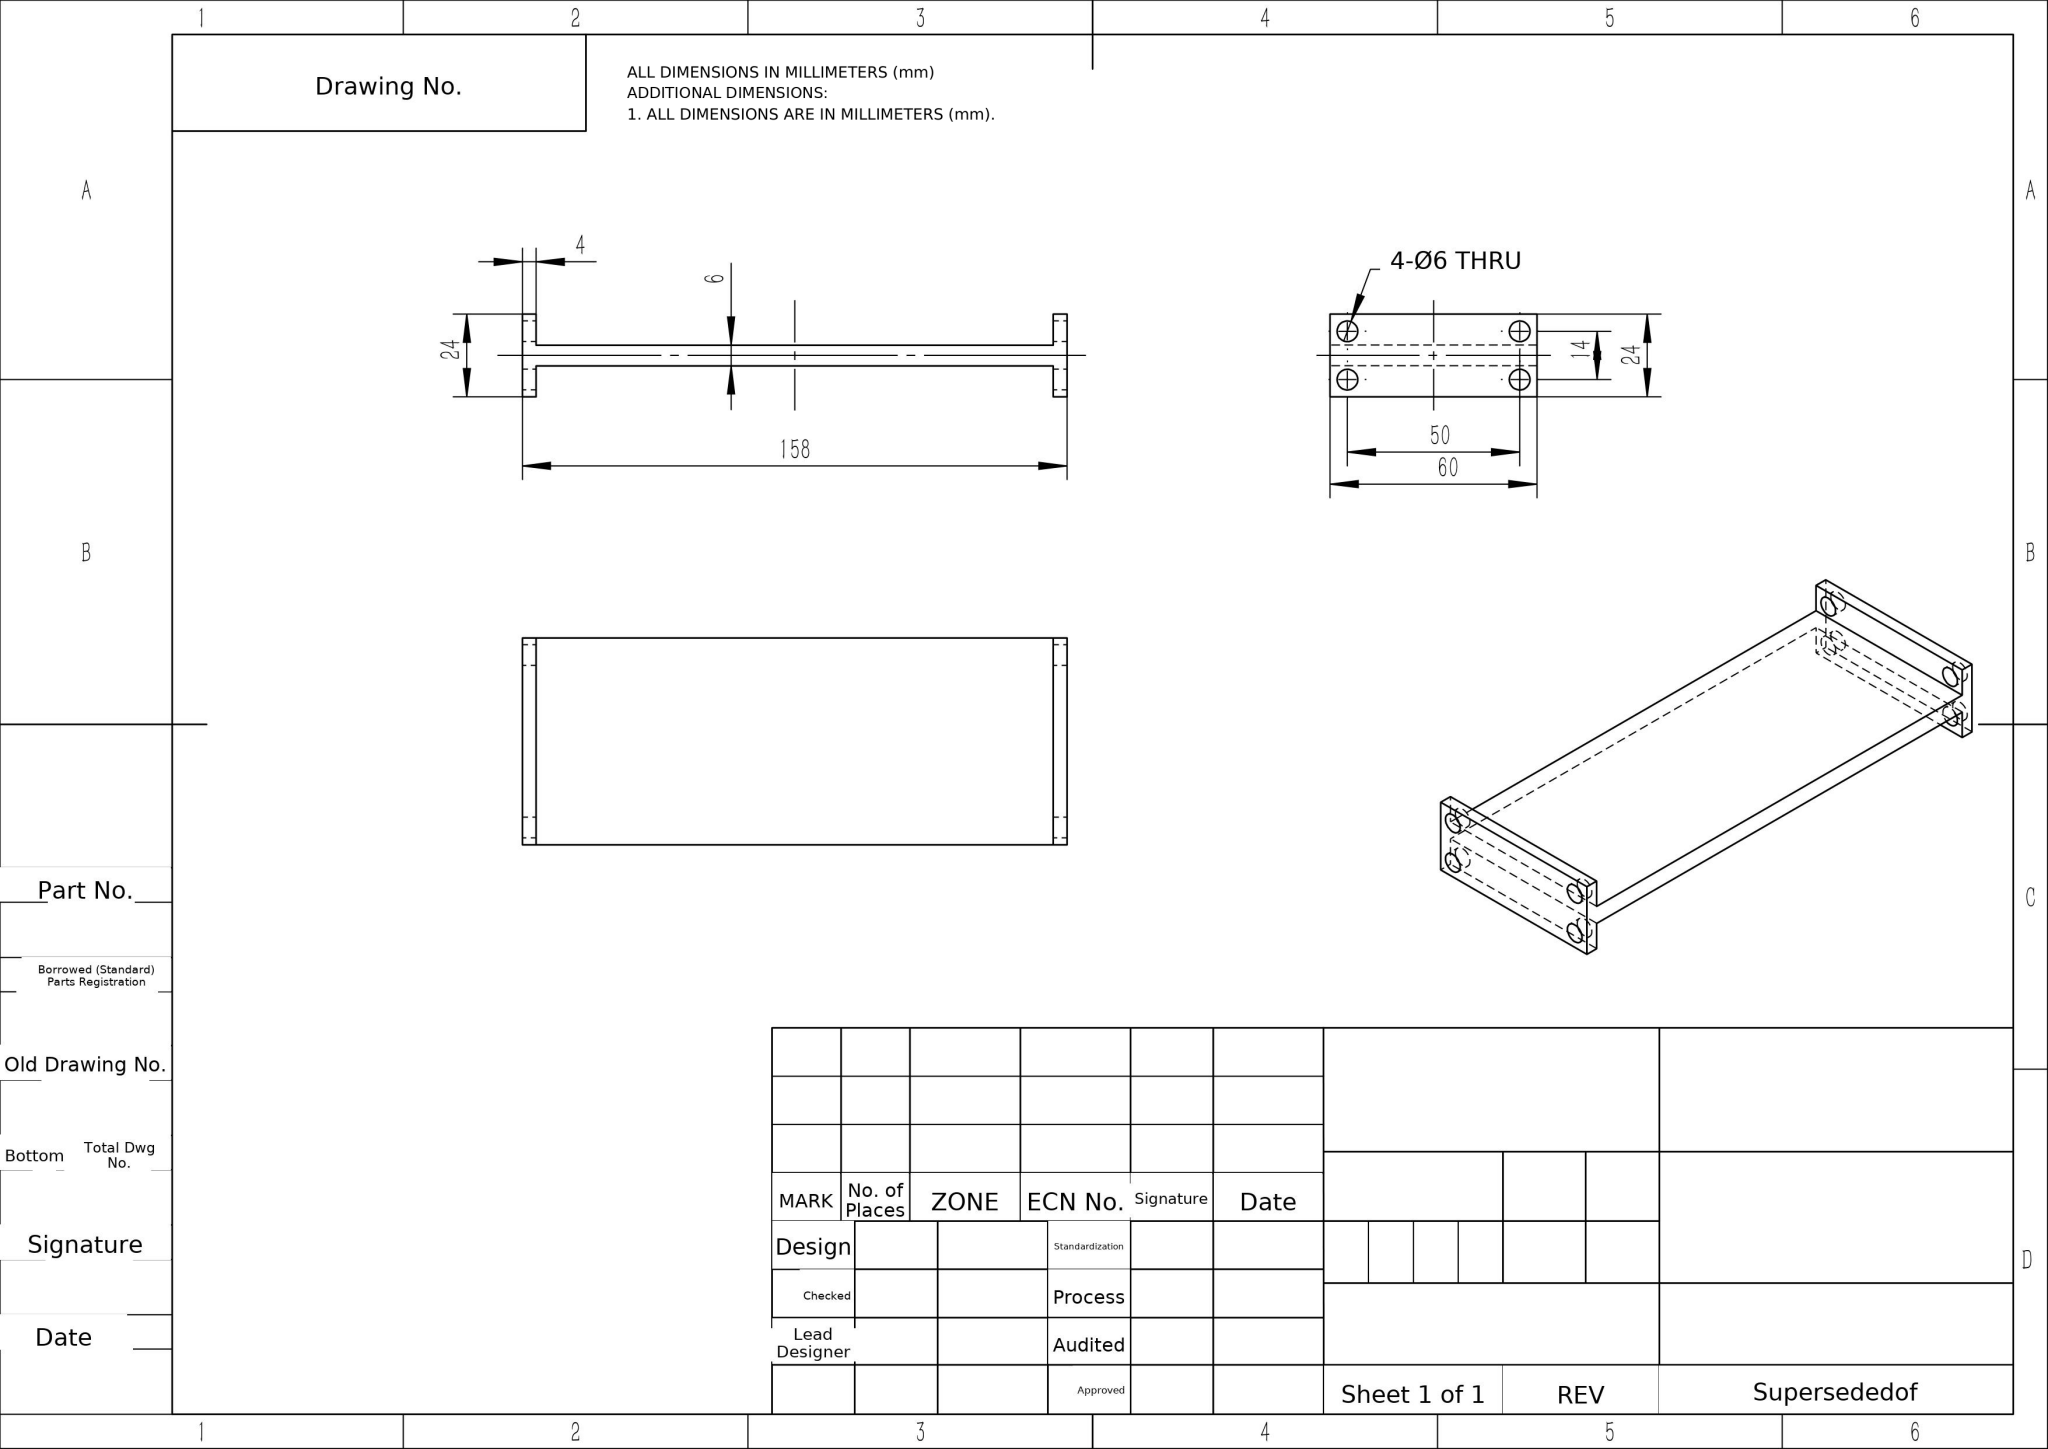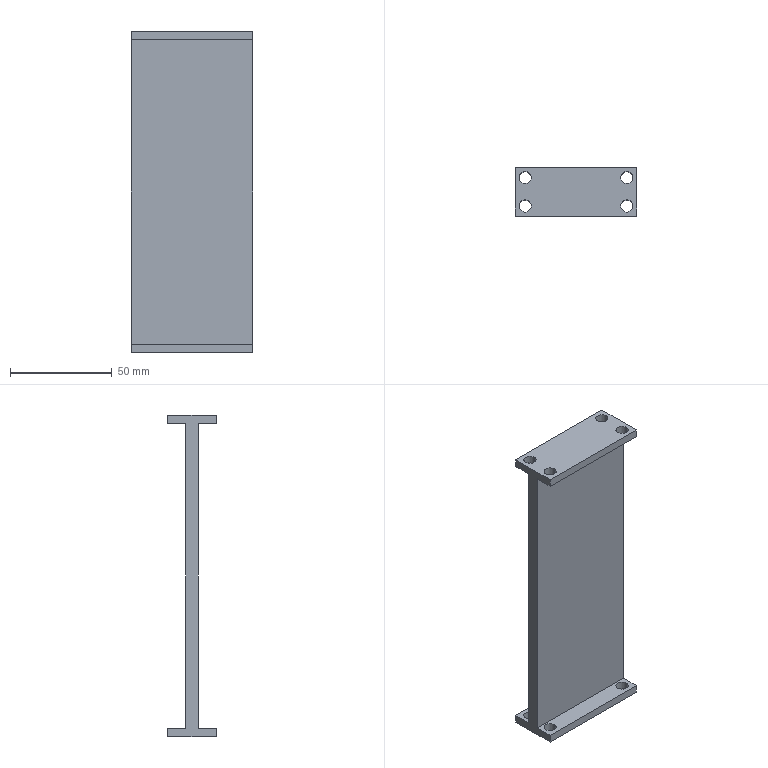Part | NX | mm | Tall Dual-Flange Panel Bracket | 1 solid | 30 faces | box 60 x 24 x 158 mm | volume 64615 mm3 | cylinder 16 | plane 14 | commonest cylinder face diameters 6 x16